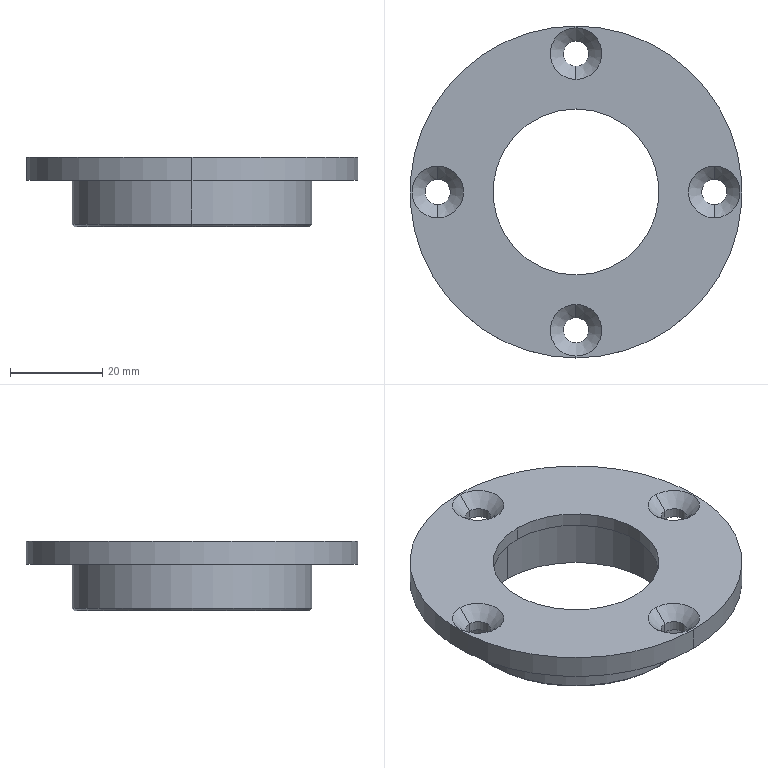Component | SolidWorks | 8TC-A15004-D0-04A-2 | 1 solid | 30 faces | box 72 x 72 x 15 mm | volume 21043 mm3 | cylinder 16 | cone 10 | plane 4 | commonest cylinder face diameters 5.5 x8 42 x2 52 x2 72 x2 36 x2 | material A3
build123d program:
from build123d import *

# Parameters (mm, degrees)
CHAMFER1_SIZE                                        = 0.5
M5_HEX_SOCKET_COUNTERSUNK_HEAD_SCREW_TAP_D           = 5.5
M5_HEX_SOCKET_COUNTERSUNK_HEAD_SCREW_TAP_CSINK_D     = 11.2
M5_HEX_SOCKET_COUNTERSUNK_HEAD_SCREW_TAP_CSINK_ANGLE = 90
CIRPATTERN1_COUNT                                    = 4


with BuildPart() as part:
    # Sketch1 → Revolve1 (revolve)
    with BuildSketch(Plane(origin=(0, 0, 0), x_dir=(1, 0, 0), z_dir=(0, 1, 0)), mode=Mode.PRIVATE) as revolve1_sk:
        Polygon((-18, 0), (-36, 0), (-36, 5), (-26, 5), (-26, 15), (-21, 15), (-21, 3), (-18, 3), align=None)
    revolve(revolve1_sk.sketch.rotate(Axis((0, 0, 0), (0, 0, -1)), 180), axis=Axis((0, 0, 0), (0, 0, -1)))

    # Chamfer1
    chamfer1_edges = [part.edges().sort_by_distance(p)[0] for p in [
        (-26, 0, -15),
    ]]
    chamfer(chamfer1_edges, length=CHAMFER1_SIZE)

    # M5 Hex Socket Countersunk Head Screw Tap (through all)
    with Locations(Plane.XY):
        with Locations((0, 30)):
            m5_hex_socket_countersunk_head_screw_tap = CounterSinkHole(M5_HEX_SOCKET_COUNTERSUNK_HEAD_SCREW_TAP_D / 2, M5_HEX_SOCKET_COUNTERSUNK_HEAD_SCREW_TAP_CSINK_D / 2, counter_sink_angle=M5_HEX_SOCKET_COUNTERSUNK_HEAD_SCREW_TAP_CSINK_ANGLE)

    # CirPattern1: M5 Hex Socket Countersunk Head Screw Tap ×4 about axis
    cirpattern1_axis = Axis((0, 0, 0), (0, 0, 1))
    for i in range(1, CIRPATTERN1_COUNT):
        add(m5_hex_socket_countersunk_head_screw_tap.rotate(cirpattern1_axis, i * 360 / CIRPATTERN1_COUNT), mode=Mode.SUBTRACT)


solid = part.part

# Placed as in the assembly
solid = solid.moved(Location((-7.5, 234.5, 125), (0, 0, 0)))
STEP:
#1=COLOUR_RGB('',0.7922,0.8196,0.9333);
#2=FILL_AREA_STYLE_COLOUR('',#1);
#3=FILL_AREA_STYLE('',(#2));
#4=SURFACE_STYLE_FILL_AREA(#3);
#5=SURFACE_SIDE_STYLE('',(#4));
#6=SURFACE_STYLE_USAGE(.BOTH.,#5);
#7=PRESENTATION_STYLE_ASSIGNMENT((#6));
#8=CARTESIAN_POINT('',(-0.2953,10.305,4.809));
#9=VERTEX_POINT('',#8);
#10=CARTESIAN_POINT('',(-0.2953,10.522,4.809));
#11=VERTEX_POINT('',#10);
#12=CARTESIAN_POINT('',(-0.2953,10.413,4.809));
#13=DIRECTION('',(0.,0.,1.));
#14=DIRECTION('',(0.,1.,0.));
#15=AXIS2_PLACEMENT_3D('',#12,#13,#14);
#16=CIRCLE('',#15,0.1083);
#17=EDGE_CURVE('',#9,#11,#16,.T.);
#18=ORIENTED_EDGE('',*,*,#17,.F.);
#19=CARTESIAN_POINT('',(-0.2953,10.193,4.921));
#20=VERTEX_POINT('',#19);
#21=CARTESIAN_POINT('',(-0.2953,10.193,4.921));
#22=DIRECTION('',(-0.,-0.7071,0.7071));
#23=VECTOR('',#22,39.37);
#24=LINE('',#21,#23);
#25=EDGE_CURVE('',#9,#20,#24,.T.);
#26=ORIENTED_EDGE('',*,*,#25,.T.);
#27=CARTESIAN_POINT('',(-0.2953,10.634,4.921));
#28=VERTEX_POINT('',#27);
#29=CARTESIAN_POINT('',(-0.2953,10.413,4.921));
#30=DIRECTION('',(0.,0.,1.));
#31=DIRECTION('',(0.,1.,0.));
#32=AXIS2_PLACEMENT_3D('',#29,#30,#31);
#33=CIRCLE('',#32,0.2205);
#34=EDGE_CURVE('',#20,#28,#33,.T.);
#35=ORIENTED_EDGE('',*,*,#34,.T.);
#36=CARTESIAN_POINT('',(-0.2953,10.634,4.921));
#37=DIRECTION('',(0.,0.7071,0.7071));
#38=VECTOR('',#37,39.37);
#39=LINE('',#36,#38);
#40=EDGE_CURVE('',#11,#28,#39,.T.);
#41=ORIENTED_EDGE('',*,*,#40,.F.);
#42=EDGE_LOOP('',(#18,#26,#35,#41));
#43=FACE_OUTER_BOUND('',#42,.T.);
#44=CARTESIAN_POINT('',(-0.2953,10.413,4.921));
#45=DIRECTION('',(0.,0.,1.));
#46=DIRECTION('',(0.,1.,0.));
#47=AXIS2_PLACEMENT_3D('',#44,#45,#46);
#48=CONICAL_SURFACE('',#47,0.2205,0.7854);
#49=ADVANCED_FACE('',(#43),#48,.F.);
#50=CARTESIAN_POINT('',(-0.2953,10.305,4.724));
#51=VERTEX_POINT('',#50);
#52=CARTESIAN_POINT('',(-0.2953,10.522,4.724));
#53=VERTEX_POINT('',#52);
#54=CARTESIAN_POINT('',(-0.2953,10.413,4.724));
#55=DIRECTION('',(0.,0.,1.));
#56=DIRECTION('',(0.,1.,0.));
#57=AXIS2_PLACEMENT_3D('',#54,#55,#56);
#58=CIRCLE('',#57,0.1083);
#59=EDGE_CURVE('',#51,#53,#58,.T.);
#60=ORIENTED_EDGE('',*,*,#59,.F.);
#61=CARTESIAN_POINT('',(-0.2953,10.305,4.921));
#62=DIRECTION('',(0.,0.,1.));
#63=VECTOR('',#62,39.37);
#64=LINE('',#61,#63);
#65=EDGE_CURVE('',#51,#9,#64,.T.);
#66=ORIENTED_EDGE('',*,*,#65,.T.);
#67=ORIENTED_EDGE('',*,*,#17,.T.);
#68=CARTESIAN_POINT('',(-0.2953,10.522,4.921));
#69=DIRECTION('',(0.,0.,1.));
#70=VECTOR('',#69,39.37);
#71=LINE('',#68,#70);
#72=EDGE_CURVE('',#53,#11,#71,.T.);
#73=ORIENTED_EDGE('',*,*,#72,.F.);
#74=EDGE_LOOP('',(#60,#66,#67,#73));
#75=FACE_OUTER_BOUND('',#74,.T.);
#76=CARTESIAN_POINT('',(-0.2953,10.413,4.921));
#77=DIRECTION('',(0.,0.,1.));
#78=DIRECTION('',(0.,1.,0.));
#79=AXIS2_PLACEMENT_3D('',#76,#77,#78);
#80=CYLINDRICAL_SURFACE('',#79,0.1083);
#81=ADVANCED_FACE('',(#75),#80,.F.);
#82=CARTESIAN_POINT('',(0.8858,9.124,4.809));
#83=VERTEX_POINT('',#82);
#84=CARTESIAN_POINT('',(0.8858,9.341,4.809));
#85=VERTEX_POINT('',#84);
#86=CARTESIAN_POINT('',(0.8858,9.232,4.809));
#87=DIRECTION('',(0.,0.,1.));
#88=DIRECTION('',(0.,1.,0.));
#89=AXIS2_PLACEMENT_3D('',#86,#87,#88);
#90=CIRCLE('',#89,0.1083);
#91=EDGE_CURVE('',#83,#85,#90,.T.);
#92=ORIENTED_EDGE('',*,*,#91,.F.);
#93=CARTESIAN_POINT('',(0.8858,9.012,4.921));
#94=VERTEX_POINT('',#93);
#95=CARTESIAN_POINT('',(0.8858,9.012,4.921));
#96=DIRECTION('',(-0.,-0.7071,0.7071));
#97=VECTOR('',#96,39.37);
#98=LINE('',#95,#97);
#99=EDGE_CURVE('',#83,#94,#98,.T.);
#100=ORIENTED_EDGE('',*,*,#99,.T.);
#101=CARTESIAN_POINT('',(0.8858,9.453,4.921));
#102=VERTEX_POINT('',#101);
#103=CARTESIAN_POINT('',(0.8858,9.232,4.921));
#104=DIRECTION('',(0.,0.,1.));
#105=DIRECTION('',(0.,1.,0.));
#106=AXIS2_PLACEMENT_3D('',#103,#104,#105);
#107=CIRCLE('',#106,0.2205);
#108=EDGE_CURVE('',#94,#102,#107,.T.);
#109=ORIENTED_EDGE('',*,*,#108,.T.);
#110=CARTESIAN_POINT('',(0.8858,9.453,4.921));
#111=DIRECTION('',(0.,0.7071,0.7071));
#112=VECTOR('',#111,39.37);
#113=LINE('',#110,#112);
#114=EDGE_CURVE('',#85,#102,#113,.T.);
#115=ORIENTED_EDGE('',*,*,#114,.F.);
#116=EDGE_LOOP('',(#92,#100,#109,#115));
#117=FACE_OUTER_BOUND('',#116,.T.);
#118=CARTESIAN_POINT('',(0.8858,9.232,4.921));
#119=DIRECTION('',(0.,0.,1.));
#120=DIRECTION('',(0.,1.,0.));
#121=AXIS2_PLACEMENT_3D('',#118,#119,#120);
#122=CONICAL_SURFACE('',#121,0.2205,0.7854);
#123=ADVANCED_FACE('',(#117),#122,.F.);
#124=CARTESIAN_POINT('',(0.8858,9.124,4.724));
#125=VERTEX_POINT('',#124);
#126=CARTESIAN_POINT('',(0.8858,9.341,4.724));
#127=VERTEX_POINT('',#126);
#128=CARTESIAN_POINT('',(0.8858,9.232,4.724));
#129=DIRECTION('',(0.,0.,1.));
#130=DIRECTION('',(0.,1.,0.));
#131=AXIS2_PLACEMENT_3D('',#128,#129,#130);
#132=CIRCLE('',#131,0.1083);
#133=EDGE_CURVE('',#125,#127,#132,.T.);
#134=ORIENTED_EDGE('',*,*,#133,.F.);
#135=CARTESIAN_POINT('',(0.8858,9.124,4.921));
#136=DIRECTION('',(0.,0.,1.));
#137=VECTOR('',#136,39.37);
#138=LINE('',#135,#137);
#139=EDGE_CURVE('',#125,#83,#138,.T.);
#140=ORIENTED_EDGE('',*,*,#139,.T.);
#141=ORIENTED_EDGE('',*,*,#91,.T.);
#142=CARTESIAN_POINT('',(0.8858,9.341,4.921));
#143=DIRECTION('',(0.,0.,1.));
#144=VECTOR('',#143,39.37);
#145=LINE('',#142,#144);
#146=EDGE_CURVE('',#127,#85,#145,.T.);
#147=ORIENTED_EDGE('',*,*,#146,.F.);
#148=EDGE_LOOP('',(#134,#140,#141,#147));
#149=FACE_OUTER_BOUND('',#148,.T.);
#150=CARTESIAN_POINT('',(0.8858,9.232,4.921));
#151=DIRECTION('',(0.,0.,1.));
#152=DIRECTION('',(0.,1.,0.));
#153=AXIS2_PLACEMENT_3D('',#150,#151,#152);
#154=CYLINDRICAL_SURFACE('',#153,0.1083);
#155=ADVANCED_FACE('',(#149),#154,.F.);
#156=CARTESIAN_POINT('',(-0.2953,7.943,4.809));
#157=VERTEX_POINT('',#156);
#158=CARTESIAN_POINT('',(-0.2953,8.159,4.809));
#159=VERTEX_POINT('',#158);
#160=CARTESIAN_POINT('',(-0.2953,8.051,4.809));
#161=DIRECTION('',(0.,0.,1.));
#162=DIRECTION('',(0.,1.,0.));
#163=AXIS2_PLACEMENT_3D('',#160,#161,#162);
#164=CIRCLE('',#163,0.1083);
#165=EDGE_CURVE('',#157,#159,#164,.T.);
#166=ORIENTED_EDGE('',*,*,#165,.F.);
#167=CARTESIAN_POINT('',(-0.2953,7.831,4.921));
#168=VERTEX_POINT('',#167);
#169=CARTESIAN_POINT('',(-0.2953,7.831,4.921));
#170=DIRECTION('',(-0.,-0.7071,0.7071));
#171=VECTOR('',#170,39.37);
#172=LINE('',#169,#171);
#173=EDGE_CURVE('',#157,#168,#172,.T.);
#174=ORIENTED_EDGE('',*,*,#173,.T.);
#175=CARTESIAN_POINT('',(-0.2953,8.272,4.921));
#176=VERTEX_POINT('',#175);
#177=CARTESIAN_POINT('',(-0.2953,8.051,4.921));
#178=DIRECTION('',(0.,0.,1.));
#179=DIRECTION('',(0.,1.,0.));
#180=AXIS2_PLACEMENT_3D('',#177,#178,#179);
#181=CIRCLE('',#180,0.2205);
#182=EDGE_CURVE('',#168,#176,#181,.T.);
#183=ORIENTED_EDGE('',*,*,#182,.T.);
#184=CARTESIAN_POINT('',(-0.2953,8.272,4.921));
#185=DIRECTION('',(0.,0.7071,0.7071));
#186=VECTOR('',#185,39.37);
#187=LINE('',#184,#186);
#188=EDGE_CURVE('',#159,#176,#187,.T.);
#189=ORIENTED_EDGE('',*,*,#188,.F.);
#190=EDGE_LOOP('',(#166,#174,#183,#189));
#191=FACE_OUTER_BOUND('',#190,.T.);
#192=CARTESIAN_POINT('',(-0.2953,8.051,4.921));
#193=DIRECTION('',(0.,0.,1.));
#194=DIRECTION('',(0.,1.,0.));
#195=AXIS2_PLACEMENT_3D('',#192,#193,#194);
#196=CONICAL_SURFACE('',#195,0.2205,0.7854);
#197=ADVANCED_FACE('',(#191),#196,.F.);
#198=CARTESIAN_POINT('',(-0.2953,7.943,4.724));
#199=VERTEX_POINT('',#198);
#200=CARTESIAN_POINT('',(-0.2953,8.159,4.724));
#201=VERTEX_POINT('',#200);
#202=CARTESIAN_POINT('',(-0.2953,8.051,4.724));
#203=DIRECTION('',(0.,0.,1.));
#204=DIRECTION('',(0.,1.,0.));
#205=AXIS2_PLACEMENT_3D('',#202,#203,#204);
#206=CIRCLE('',#205,0.1083);
#207=EDGE_CURVE('',#199,#201,#206,.T.);
#208=ORIENTED_EDGE('',*,*,#207,.F.);
#209=CARTESIAN_POINT('',(-0.2953,7.943,4.921));
#210=DIRECTION('',(0.,0.,1.));
#211=VECTOR('',#210,39.37);
#212=LINE('',#209,#211);
#213=EDGE_CURVE('',#199,#157,#212,.T.);
#214=ORIENTED_EDGE('',*,*,#213,.T.);
#215=ORIENTED_EDGE('',*,*,#165,.T.);
#216=CARTESIAN_POINT('',(-0.2953,8.159,4.921));
#217=DIRECTION('',(0.,0.,1.));
#218=VECTOR('',#217,39.37);
#219=LINE('',#216,#218);
#220=EDGE_CURVE('',#201,#159,#219,.T.);
#221=ORIENTED_EDGE('',*,*,#220,.F.);
#222=EDGE_LOOP('',(#208,#214,#215,#221));
#223=FACE_OUTER_BOUND('',#222,.T.);
#224=CARTESIAN_POINT('',(-0.2953,8.051,4.921));
#225=DIRECTION('',(0.,0.,1.));
#226=DIRECTION('',(0.,1.,0.));
#227=AXIS2_PLACEMENT_3D('',#224,#225,#226);
#228=CYLINDRICAL_SURFACE('',#227,0.1083);
#229=ADVANCED_FACE('',(#223),#228,.F.);
#230=CARTESIAN_POINT('',(-1.476,9.124,4.809));
#231=VERTEX_POINT('',#230);
#232=CARTESIAN_POINT('',(-1.476,9.341,4.809));
#233=VERTEX_POINT('',#232);
#234=CARTESIAN_POINT('',(-1.476,9.232,4.809));
#235=DIRECTION('',(0.,0.,1.));
#236=DIRECTION('',(0.,1.,0.));
#237=AXIS2_PLACEMENT_3D('',#234,#235,#236);
#238=CIRCLE('',#237,0.1083);
#239=EDGE_CURVE('',#231,#233,#238,.T.);
#240=ORIENTED_EDGE('',*,*,#239,.F.);
#241=CARTESIAN_POINT('',(-1.476,9.012,4.921));
#242=VERTEX_POINT('',#241);
#243=CARTESIAN_POINT('',(-1.476,9.012,4.921));
#244=DIRECTION('',(-0.,-0.7071,0.7071));
#245=VECTOR('',#244,39.37);
#246=LINE('',#243,#245);
#247=EDGE_CURVE('',#231,#242,#246,.T.);
#248=ORIENTED_EDGE('',*,*,#247,.T.);
#249=CARTESIAN_POINT('',(-1.476,9.453,4.921));
#250=VERTEX_POINT('',#249);
#251=CARTESIAN_POINT('',(-1.476,9.232,4.921));
#252=DIRECTION('',(0.,0.,1.));
#253=DIRECTION('',(0.,1.,0.));
#254=AXIS2_PLACEMENT_3D('',#251,#252,#253);
#255=CIRCLE('',#254,0.2205);
#256=EDGE_CURVE('',#242,#250,#255,.T.);
#257=ORIENTED_EDGE('',*,*,#256,.T.);
#258=CARTESIAN_POINT('',(-1.476,9.453,4.921));
#259=DIRECTION('',(0.,0.7071,0.7071));
#260=VECTOR('',#259,39.37);
#261=LINE('',#258,#260);
#262=EDGE_CURVE('',#233,#250,#261,.T.);
#263=ORIENTED_EDGE('',*,*,#262,.F.);
#264=EDGE_LOOP('',(#240,#248,#257,#263));
#265=FACE_OUTER_BOUND('',#264,.T.);
#266=CARTESIAN_POINT('',(-1.476,9.232,4.921));
#267=DIRECTION('',(0.,0.,1.));
#268=DIRECTION('',(0.,1.,0.));
#269=AXIS2_PLACEMENT_3D('',#266,#267,#268);
#270=CONICAL_SURFACE('',#269,0.2205,0.7854);
#271=ADVANCED_FACE('',(#265),#270,.F.);
#272=CARTESIAN_POINT('',(-1.476,9.124,4.724));
#273=VERTEX_POINT('',#272);
#274=CARTESIAN_POINT('',(-1.476,9.341,4.724));
#275=VERTEX_POINT('',#274);
#276=CARTESIAN_POINT('',(-1.476,9.232,4.724));
#277=DIRECTION('',(0.,0.,1.));
#278=DIRECTION('',(0.,1.,0.));
#279=AXIS2_PLACEMENT_3D('',#276,#277,#278);
#280=CIRCLE('',#279,0.1083);
#281=EDGE_CURVE('',#273,#275,#280,.T.);
#282=ORIENTED_EDGE('',*,*,#281,.F.);
#283=CARTESIAN_POINT('',(-1.476,9.124,4.921));
#284=DIRECTION('',(0.,0.,1.));
#285=VECTOR('',#284,39.37);
#286=LINE('',#283,#285);
#287=EDGE_CURVE('',#273,#231,#286,.T.);
#288=ORIENTED_EDGE('',*,*,#287,.T.);
#289=ORIENTED_EDGE('',*,*,#239,.T.);
#290=CARTESIAN_POINT('',(-1.476,9.341,4.921));
#291=DIRECTION('',(0.,0.,1.));
#292=VECTOR('',#291,39.37);
#293=LINE('',#290,#292);
#294=EDGE_CURVE('',#275,#233,#293,.T.);
#295=ORIENTED_EDGE('',*,*,#294,.F.);
#296=EDGE_LOOP('',(#282,#288,#289,#295));
#297=FACE_OUTER_BOUND('',#296,.T.);
#298=CARTESIAN_POINT('',(-1.476,9.232,4.921));
#299=DIRECTION('',(0.,0.,1.));
#300=DIRECTION('',(0.,1.,0.));
#301=AXIS2_PLACEMENT_3D('',#298,#299,#300);
#302=CYLINDRICAL_SURFACE('',#301,0.1083);
#303=ADVANCED_FACE('',(#297),#302,.F.);
#304=CARTESIAN_POINT('',(-0.2953,8.228,4.331));
#305=VERTEX_POINT('',#304);
#306=CARTESIAN_POINT('',(-0.2953,10.236,4.331));
#307=VERTEX_POINT('',#306);
#308=CARTESIAN_POINT('',(-0.2953,9.232,4.331));
#309=DIRECTION('',(0.,0.,-1.));
#310=DIRECTION('',(0.,1.,0.));
#311=AXIS2_PLACEMENT_3D('',#308,#309,#310);
#312=CIRCLE('',#311,1.004);
#313=EDGE_CURVE('',#305,#307,#312,.T.);
#314=ORIENTED_EDGE('',*,*,#313,.F.);
#315=CARTESIAN_POINT('',(-0.2953,8.209,4.35));
#316=VERTEX_POINT('',#315);
#317=CARTESIAN_POINT('',(-0.2953,8.209,4.35));
#318=DIRECTION('',(-0.,-0.7071,0.7071));
#319=VECTOR('',#318,39.37);
#320=LINE('',#317,#319);
#321=EDGE_CURVE('',#305,#316,#320,.T.);
#322=ORIENTED_EDGE('',*,*,#321,.T.);
#323=CARTESIAN_POINT('',(-0.2953,10.256,4.35));
#324=VERTEX_POINT('',#323);
#325=CARTESIAN_POINT('',(-0.2953,9.232,4.35));
#326=DIRECTION('',(0.,0.,1.));
#327=DIRECTION('',(0.,1.,0.));
#328=AXIS2_PLACEMENT_3D('',#325,#326,#327);
#329=CIRCLE('',#328,1.024);
#330=EDGE_CURVE('',#324,#316,#329,.T.);
#331=ORIENTED_EDGE('',*,*,#330,.F.);
#332=CARTESIAN_POINT('',(-0.2953,10.256,4.35));
#333=DIRECTION('',(0.,0.7071,0.7071));
#334=VECTOR('',#333,39.37);
#335=LINE('',#332,#334);
#336=EDGE_CURVE('',#307,#324,#335,.T.);
#337=ORIENTED_EDGE('',*,*,#336,.F.);
#338=EDGE_LOOP('',(#314,#322,#331,#337));
#339=FACE_OUTER_BOUND('',#338,.T.);
#340=CARTESIAN_POINT('',(-0.2953,9.232,4.35));
#341=DIRECTION('',(0.,0.,1.));
#342=DIRECTION('',(0.,1.,0.));
#343=AXIS2_PLACEMENT_3D('',#340,#341,#342);
#344=CONICAL_SURFACE('',#343,1.024,0.7854);
#345=ADVANCED_FACE('',(#339),#344,.T.);
#346=CARTESIAN_POINT('',(-0.2953,8.406,4.331));
#347=VERTEX_POINT('',#346);
#348=CARTESIAN_POINT('',(-0.2953,10.059,4.331));
#349=VERTEX_POINT('',#348);
#350=CARTESIAN_POINT('',(-0.2953,9.232,4.331));
#351=DIRECTION('',(0.,0.,1.));
#352=DIRECTION('',(0.,1.,0.));
#353=AXIS2_PLACEMENT_3D('',#350,#351,#352);
#354=CIRCLE('',#353,0.8268);
#355=EDGE_CURVE('',#347,#349,#354,.T.);
#356=ORIENTED_EDGE('',*,*,#355,.F.);
#357=CARTESIAN_POINT('',(-0.2953,8.406,4.803));
#358=VERTEX_POINT('',#357);
#359=CARTESIAN_POINT('',(-0.2953,8.406,4.921));
#360=DIRECTION('',(0.,0.,1.));
#361=VECTOR('',#360,39.37);
#362=LINE('',#359,#361);
#363=EDGE_CURVE('',#347,#358,#362,.T.);
#364=ORIENTED_EDGE('',*,*,#363,.T.);
#365=CARTESIAN_POINT('',(-0.2953,10.059,4.803));
#366=VERTEX_POINT('',#365);
#367=CARTESIAN_POINT('',(-0.2953,9.232,4.803));
#368=DIRECTION('',(0.,0.,1.));
#369=DIRECTION('',(0.,1.,0.));
#370=AXIS2_PLACEMENT_3D('',#367,#368,#369);
#371=CIRCLE('',#370,0.8268);
#372=EDGE_CURVE('',#358,#366,#371,.T.);
#373=ORIENTED_EDGE('',*,*,#372,.T.);
#374=CARTESIAN_POINT('',(-0.2953,10.059,4.921));
#375=DIRECTION('',(0.,0.,1.));
#376=VECTOR('',#375,39.37);
#377=LINE('',#374,#376);
#378=EDGE_CURVE('',#349,#366,#377,.T.);
#379=ORIENTED_EDGE('',*,*,#378,.F.);
#380=EDGE_LOOP('',(#356,#364,#373,#379));
#381=FACE_OUTER_BOUND('',#380,.T.);
#382=CARTESIAN_POINT('',(-0.2953,9.232,4.921));
#383=DIRECTION('',(0.,0.,1.));
#384=DIRECTION('',(0.,1.,0.));
#385=AXIS2_PLACEMENT_3D('',#382,#383,#384);
#386=CYLINDRICAL_SURFACE('',#385,0.8268);
#387=ADVANCED_FACE('',(#381),#386,.F.);
#388=ORIENTED_EDGE('',*,*,#330,.T.);
#389=CARTESIAN_POINT('',(-0.2953,8.209,4.724));
#390=VERTEX_POINT('',#389);
#391=CARTESIAN_POINT('',(-0.2953,8.209,4.921));
#392=DIRECTION('',(0.,0.,1.));
#393=VECTOR('',#392,39.37);
#394=LINE('',#391,#393);
#395=EDGE_CURVE('',#316,#390,#394,.T.);
#396=ORIENTED_EDGE('',*,*,#395,.T.);
#397=CARTESIAN_POINT('',(-0.2953,10.256,4.724));
#398=VERTEX_POINT('',#397);
#399=CARTESIAN_POINT('',(-0.2953,9.232,4.724));
#400=DIRECTION('',(0.,0.,1.));
#401=DIRECTION('',(0.,1.,0.));
#402=AXIS2_PLACEMENT_3D('',#399,#400,#401);
#403=CIRCLE('',#402,1.024);
#404=EDGE_CURVE('',#398,#390,#403,.T.);
#405=ORIENTED_EDGE('',*,*,#404,.F.);
#406=CARTESIAN_POINT('',(-0.2953,10.256,4.921));
#407=DIRECTION('',(0.,0.,1.));
#408=VECTOR('',#407,39.37);
#409=LINE('',#406,#408);
#410=EDGE_CURVE('',#324,#398,#409,.T.);
#411=ORIENTED_EDGE('',*,*,#410,.F.);
#412=EDGE_LOOP('',(#388,#396,#405,#411));
#413=FACE_OUTER_BOUND('',#412,.T.);
#414=CARTESIAN_POINT('',(-0.2953,9.232,4.921));
#415=DIRECTION('',(0.,0.,1.));
#416=DIRECTION('',(0.,1.,0.));
#417=AXIS2_PLACEMENT_3D('',#414,#415,#416);
#418=CYLINDRICAL_SURFACE('',#417,1.024);
#419=ADVANCED_FACE('',(#413),#418,.T.);
#420=CARTESIAN_POINT('',(-0.2953,10.65,4.724));
#421=VERTEX_POINT('',#420);
#422=CARTESIAN_POINT('',(-0.2953,7.815,4.724));
#423=VERTEX_POINT('',#422);
#424=CARTESIAN_POINT('',(-0.2953,9.232,4.724));
#425=DIRECTION('',(0.,0.,1.));
#426=DIRECTION('',(0.,1.,0.));
#427=AXIS2_PLACEMENT_3D('',#424,#425,#426);
#428=CIRCLE('',#427,1.417);
#429=EDGE_CURVE('',#421,#423,#428,.T.);
#430=ORIENTED_EDGE('',*,*,#429,.T.);
#431=CARTESIAN_POINT('',(-0.2953,7.815,4.921));
#432=VERTEX_POINT('',#431);
#433=CARTESIAN_POINT('',(-0.2953,7.815,4.921));
#434=DIRECTION('',(0.,0.,1.));
#435=VECTOR('',#434,39.37);
#436=LINE('',#433,#435);
#437=EDGE_CURVE('',#423,#432,#436,.T.);
#438=ORIENTED_EDGE('',*,*,#437,.T.);
#439=CARTESIAN_POINT('',(-0.2953,10.65,4.921));
#440=VERTEX_POINT('',#439);
#441=CARTESIAN_POINT('',(-0.2953,9.232,4.921));
#442=DIRECTION('',(0.,0.,1.));
#443=DIRECTION('',(0.,1.,0.));
#444=AXIS2_PLACEMENT_3D('',#441,#442,#443);
#445=CIRCLE('',#444,1.417);
#446=EDGE_CURVE('',#440,#432,#445,.T.);
#447=ORIENTED_EDGE('',*,*,#446,.F.);
#448=CARTESIAN_POINT('',(-0.2953,10.65,4.921));
#449=DIRECTION('',(0.,0.,1.));
#450=VECTOR('',#449,39.37);
#451=LINE('',#448,#450);
#452=EDGE_CURVE('',#421,#440,#451,.T.);
#453=ORIENTED_EDGE('',*,*,#452,.F.);
#454=EDGE_LOOP('',(#430,#438,#447,#453));
#455=FACE_OUTER_BOUND('',#454,.T.);
#456=CARTESIAN_POINT('',(-0.2953,9.232,4.921));
#457=DIRECTION('',(0.,0.,1.));
#458=DIRECTION('',(0.,1.,0.));
#459=AXIS2_PLACEMENT_3D('',#456,#457,#458);
#460=CYLINDRICAL_SURFACE('',#459,1.417);
#461=ADVANCED_FACE('',(#455),#460,.T.);
#462=CARTESIAN_POINT('',(-0.2953,8.524,4.803));
#463=VERTEX_POINT('',#462);
#464=CARTESIAN_POINT('',(-0.2953,9.941,4.803));
#465=VERTEX_POINT('',#464);
#466=CARTESIAN_POINT('',(-0.2953,9.232,4.803));
#467=DIRECTION('',(0.,0.,1.));
#468=DIRECTION('',(0.,1.,0.));
#469=AXIS2_PLACEMENT_3D('',#466,#467,#468);
#470=CIRCLE('',#469,0.7087);
#471=EDGE_CURVE('',#463,#465,#470,.T.);
#472=ORIENTED_EDGE('',*,*,#471,.F.);
#473=CARTESIAN_POINT('',(-0.2953,8.524,4.921));
#474=VERTEX_POINT('',#473);
#475=CARTESIAN_POINT('',(-0.2953,8.524,4.921));
#476=DIRECTION('',(0.,0.,1.));
#477=VECTOR('',#476,39.37);
#478=LINE('',#475,#477);
#479=EDGE_CURVE('',#463,#474,#478,.T.);
#480=ORIENTED_EDGE('',*,*,#479,.T.);
#481=CARTESIAN_POINT('',(-0.2953,9.941,4.921));
#482=VERTEX_POINT('',#481);
#483=CARTESIAN_POINT('',(-0.2953,9.232,4.921));
#484=DIRECTION('',(0.,0.,1.));
#485=DIRECTION('',(0.,1.,0.));
#486=AXIS2_PLACEMENT_3D('',#483,#484,#485);
#487=CIRCLE('',#486,0.7087);
#488=EDGE_CURVE('',#474,#482,#487,.T.);
#489=ORIENTED_EDGE('',*,*,#488,.T.);
#490=CARTESIAN_POINT('',(-0.2953,9.941,4.921));
#491=DIRECTION('',(0.,0.,1.));
#492=VECTOR('',#491,39.37);
#493=LINE('',#490,#492);
#494=EDGE_CURVE('',#465,#482,#493,.T.);
#495=ORIENTED_EDGE('',*,*,#494,.F.);
#496=EDGE_LOOP('',(#472,#480,#489,#495));
#497=FACE_OUTER_BOUND('',#496,.T.);
#498=CARTESIAN_POINT('',(-0.2953,9.232,4.921));
#499=DIRECTION('',(0.,0.,1.));
#500=DIRECTION('',(0.,1.,0.));
#501=AXIS2_PLACEMENT_3D('',#498,#499,#500);
#502=CYLINDRICAL_SURFACE('',#501,0.7087);
#503=ADVANCED_FACE('',(#497),#502,.F.);
#504=ORIENTED_EDGE('',*,*,#479,.F.);
#505=CARTESIAN_POINT('',(-0.2953,9.232,4.803));
#506=DIRECTION('',(0.,0.,1.));
#507=DIRECTION('',(0.,1.,0.));
#508=AXIS2_PLACEMENT_3D('',#505,#506,#507);
#509=CIRCLE('',#508,0.7087);
#510=EDGE_CURVE('',#465,#463,#509,.T.);
#511=ORIENTED_EDGE('',*,*,#510,.F.);
#512=ORIENTED_EDGE('',*,*,#494,.T.);
#513=CARTESIAN_POINT('',(-0.2953,9.232,4.921));
#514=DIRECTION('',(0.,0.,1.));
#515=DIRECTION('',(0.,1.,0.));
#516=AXIS2_PLACEMENT_3D('',#513,#514,#515);
#517=CIRCLE('',#516,0.7087);
#518=EDGE_CURVE('',#482,#474,#517,.T.);
#519=ORIENTED_EDGE('',*,*,#518,.T.);
#520=EDGE_LOOP('',(#504,#511,#512,#519));
#521=FACE_OUTER_BOUND('',#520,.T.);
#522=CARTESIAN_POINT('',(-0.2953,9.232,4.921));
#523=DIRECTION('',(0.,0.,1.));
#524=DIRECTION('',(0.,1.,0.));
#525=AXIS2_PLACEMENT_3D('',#522,#523,#524);
#526=CYLINDRICAL_SURFACE('',#525,0.7087);
#527=ADVANCED_FACE('',(#521),#526,.F.);
#528=CARTESIAN_POINT('',(-0.2953,10.413,4.921));
#529=DIRECTION('',(0.,0.,1.));
#530=DIRECTION('',(0.,1.,0.));
#531=AXIS2_PLACEMENT_3D('',#528,#529,#530);
#532=CIRCLE('',#531,0.2205);
#533=EDGE_CURVE('',#28,#20,#532,.T.);
#534=ORIENTED_EDGE('',*,*,#533,.F.);
#535=ORIENTED_EDGE('',*,*,#34,.F.);
#536=EDGE_LOOP('',(#534,#535));
#537=FACE_BOUND('',#536,.T.);
#538=CARTESIAN_POINT('',(0.8858,9.232,4.921));
#539=DIRECTION('',(0.,0.,1.));
#540=DIRECTION('',(0.,1.,0.));
#541=AXIS2_PLACEMENT_3D('',#538,#539,#540);
#542=CIRCLE('',#541,0.2205);
#543=EDGE_CURVE('',#102,#94,#542,.T.);
#544=ORIENTED_EDGE('',*,*,#543,.F.);
#545=ORIENTED_EDGE('',*,*,#108,.F.);
#546=EDGE_LOOP('',(#544,#545));
#547=FACE_BOUND('',#546,.T.);
#548=CARTESIAN_POINT('',(-0.2953,8.051,4.921));
#549=DIRECTION('',(0.,0.,1.));
#550=DIRECTION('',(0.,1.,0.));
#551=AXIS2_PLACEMENT_3D('',#548,#549,#550);
#552=CIRCLE('',#551,0.2205);
#553=EDGE_CURVE('',#176,#168,#552,.T.);
#554=ORIENTED_EDGE('',*,*,#553,.F.);
#555=ORIENTED_EDGE('',*,*,#182,.F.);
#556=EDGE_LOOP('',(#554,#555));
#557=FACE_BOUND('',#556,.T.);
#558=CARTESIAN_POINT('',(-1.476,9.232,4.921));
#559=DIRECTION('',(0.,0.,1.));
#560=DIRECTION('',(0.,1.,0.));
#561=AXIS2_PLACEMENT_3D('',#558,#559,#560);
#562=CIRCLE('',#561,0.2205);
#563=EDGE_CURVE('',#250,#242,#562,.T.);
#564=ORIENTED_EDGE('',*,*,#563,.F.);
#565=ORIENTED_EDGE('',*,*,#256,.F.);
#566=EDGE_LOOP('',(#564,#565));
#567=FACE_BOUND('',#566,.T.);
#568=ORIENTED_EDGE('',*,*,#518,.F.);
#569=ORIENTED_EDGE('',*,*,#488,.F.);
#570=EDGE_LOOP('',(#568,#569));
#571=FACE_BOUND('',#570,.T.);
#572=ORIENTED_EDGE('',*,*,#446,.T.);
#573=CARTESIAN_POINT('',(-0.2953,9.232,4.921));
#574=DIRECTION('',(0.,0.,1.));
#575=DIRECTION('',(0.,1.,0.));
#576=AXIS2_PLACEMENT_3D('',#573,#574,#575);
#577=CIRCLE('',#576,1.417);
#578=EDGE_CURVE('',#432,#440,#577,.T.);
#579=ORIENTED_EDGE('',*,*,#578,.T.);
#580=EDGE_LOOP('',(#572,#579));
#581=FACE_OUTER_BOUND('',#580,.T.);
#582=CARTESIAN_POINT('',(-0.2953,8.524,4.921));
#583=DIRECTION('',(0.,0.,-1.));
#584=DIRECTION('',(-0.,-1.,0.));
#585=AXIS2_PLACEMENT_3D('',#582,#583,#584);
#586=PLANE('',#585);
#587=ADVANCED_FACE('',(#537,#547,#557,#567,#571,#581),#586,.F.);
#588=ORIENTED_EDGE('',*,*,#437,.F.);
#589=CARTESIAN_POINT('',(-0.2953,9.232,4.724));
#590=DIRECTION('',(0.,0.,1.));
#591=DIRECTION('',(0.,1.,0.));
#592=AXIS2_PLACEMENT_3D('',#589,#590,#591);
#593=CIRCLE('',#592,1.417);
#594=EDGE_CURVE('',#423,#421,#593,.T.);
#595=ORIENTED_EDGE('',*,*,#594,.T.);
#596=ORIENTED_EDGE('',*,*,#452,.T.);
#597=ORIENTED_EDGE('',*,*,#578,.F.);
#598=EDGE_LOOP('',(#588,#595,#596,#597));
#599=FACE_OUTER_BOUND('',#598,.T.);
#600=CARTESIAN_POINT('',(-0.2953,9.232,4.921));
#601=DIRECTION('',(0.,0.,1.));
#602=DIRECTION('',(0.,1.,0.));
#603=AXIS2_PLACEMENT_3D('',#600,#601,#602);
#604=CYLINDRICAL_SURFACE('',#603,1.417);
#605=ADVANCED_FACE('',(#599),#604,.T.);
#606=CARTESIAN_POINT('',(-0.2953,10.413,4.724));
#607=DIRECTION('',(0.,0.,1.));
#608=DIRECTION('',(0.,1.,0.));
#609=AXIS2_PLACEMENT_3D('',#606,#607,#608);
#610=CIRCLE('',#609,0.1083);
#611=EDGE_CURVE('',#53,#51,#610,.T.);
#612=ORIENTED_EDGE('',*,*,#611,.T.);
#613=ORIENTED_EDGE('',*,*,#59,.T.);
#614=EDGE_LOOP('',(#612,#613));
#615=FACE_BOUND('',#614,.T.);
#616=CARTESIAN_POINT('',(0.8858,9.232,4.724));
#617=DIRECTION('',(0.,0.,1.));
#618=DIRECTION('',(0.,1.,0.));
#619=AXIS2_PLACEMENT_3D('',#616,#617,#618);
#620=CIRCLE('',#619,0.1083);
#621=EDGE_CURVE('',#127,#125,#620,.T.);
#622=ORIENTED_EDGE('',*,*,#621,.T.);
#623=ORIENTED_EDGE('',*,*,#133,.T.);
#624=EDGE_LOOP('',(#622,#623));
#625=FACE_BOUND('',#624,.T.);
#626=CARTESIAN_POINT('',(-0.2953,8.051,4.724));
#627=DIRECTION('',(0.,0.,1.));
#628=DIRECTION('',(0.,1.,0.));
#629=AXIS2_PLACEMENT_3D('',#626,#627,#628);
#630=CIRCLE('',#629,0.1083);
#631=EDGE_CURVE('',#201,#199,#630,.T.);
#632=ORIENTED_EDGE('',*,*,#631,.T.);
#633=ORIENTED_EDGE('',*,*,#207,.T.);
#634=EDGE_LOOP('',(#632,#633));
#635=FACE_BOUND('',#634,.T.);
#636=CARTESIAN_POINT('',(-1.476,9.232,4.724));
#637=DIRECTION('',(0.,0.,1.));
#638=DIRECTION('',(0.,1.,0.));
#639=AXIS2_PLACEMENT_3D('',#636,#637,#638);
#640=CIRCLE('',#639,0.1083);
#641=EDGE_CURVE('',#275,#273,#640,.T.);
#642=ORIENTED_EDGE('',*,*,#641,.T.);
#643=ORIENTED_EDGE('',*,*,#281,.T.);
#644=EDGE_LOOP('',(#642,#643));
#645=FACE_BOUND('',#644,.T.);
#646=ORIENTED_EDGE('',*,*,#429,.F.);
#647=ORIENTED_EDGE('',*,*,#594,.F.);
#648=EDGE_LOOP('',(#646,#647));
#649=FACE_OUTER_BOUND('',#648,.T.);
#650=ORIENTED_EDGE('',*,*,#404,.T.);
#651=CARTESIAN_POINT('',(-0.2953,9.232,4.724));
#652=DIRECTION('',(0.,0.,1.));
#653=DIRECTION('',(0.,1.,0.));
#654=AXIS2_PLACEMENT_3D('',#651,#652,#653);
#655=CIRCLE('',#654,1.024);
#656=EDGE_CURVE('',#390,#398,#655,.T.);
#657=ORIENTED_EDGE('',*,*,#656,.T.);
#658=EDGE_LOOP('',(#650,#657));
#659=FACE_BOUND('',#658,.T.);
#660=CARTESIAN_POINT('',(-0.2953,7.815,4.724));
#661=DIRECTION('',(0.,0.,1.));
#662=DIRECTION('',(0.,1.,0.));
#663=AXIS2_PLACEMENT_3D('',#660,#661,#662);
#664=PLANE('',#663);
#665=ADVANCED_FACE('',(#615,#625,#635,#645,#649,#659),#664,.F.);
#666=ORIENTED_EDGE('',*,*,#395,.F.);
#667=CARTESIAN_POINT('',(-0.2953,9.232,4.35));
#668=DIRECTION('',(0.,0.,1.));
#669=DIRECTION('',(0.,1.,0.));
#670=AXIS2_PLACEMENT_3D('',#667,#668,#669);
#671=CIRCLE('',#670,1.024);
#672=EDGE_CURVE('',#316,#324,#671,.T.);
#673=ORIENTED_EDGE('',*,*,#672,.T.);
#674=ORIENTED_EDGE('',*,*,#410,.T.);
#675=ORIENTED_EDGE('',*,*,#656,.F.);
#676=EDGE_LOOP('',(#666,#673,#674,#675));
#677=FACE_OUTER_BOUND('',#676,.T.);
#678=CARTESIAN_POINT('',(-0.2953,9.232,4.921));
#679=DIRECTION('',(0.,0.,1.));
#680=DIRECTION('',(0.,1.,0.));
#681=AXIS2_PLACEMENT_3D('',#678,#679,#680);
#682=CYLINDRICAL_SURFACE('',#681,1.024);
#683=ADVANCED_FACE('',(#677),#682,.T.);
#684=CARTESIAN_POINT('',(-0.2953,9.232,4.331));
#685=DIRECTION('',(0.,0.,-1.));
#686=DIRECTION('',(0.,1.,0.));
#687=AXIS2_PLACEMENT_3D('',#684,#685,#686);
#688=CIRCLE('',#687,1.004);
#689=EDGE_CURVE('',#307,#305,#688,.T.);
#690=ORIENTED_EDGE('',*,*,#689,.T.);
#691=ORIENTED_EDGE('',*,*,#313,.T.);
#692=EDGE_LOOP('',(#690,#691));
#693=FACE_OUTER_BOUND('',#692,.T.);
#694=CARTESIAN_POINT('',(-0.2953,9.232,4.331));
#695=DIRECTION('',(0.,0.,1.));
#696=DIRECTION('',(0.,1.,0.));
#697=AXIS2_PLACEMENT_3D('',#694,#695,#696);
#698=CIRCLE('',#697,0.8268);
#699=EDGE_CURVE('',#349,#347,#698,.T.);
#700=ORIENTED_EDGE('',*,*,#699,.T.);
#701=ORIENTED_EDGE('',*,*,#355,.T.);
#702=EDGE_LOOP('',(#700,#701));
#703=FACE_BOUND('',#702,.T.);
#704=CARTESIAN_POINT('',(-0.2953,8.209,4.331));
#705=DIRECTION('',(0.,0.,1.));
#706=DIRECTION('',(0.,1.,0.));
#707=AXIS2_PLACEMENT_3D('',#704,#705,#706);
#708=PLANE('',#707);
#709=ADVANCED_FACE('',(#693,#703),#708,.F.);
#710=ORIENTED_EDGE('',*,*,#363,.F.);
#711=ORIENTED_EDGE('',*,*,#699,.F.);
#712=ORIENTED_EDGE('',*,*,#378,.T.);
#713=CARTESIAN_POINT('',(-0.2953,9.232,4.803));
#714=DIRECTION('',(0.,0.,1.));
#715=DIRECTION('',(0.,1.,0.));
#716=AXIS2_PLACEMENT_3D('',#713,#714,#715);
#717=CIRCLE('',#716,0.8268);
#718=EDGE_CURVE('',#366,#358,#717,.T.);
#719=ORIENTED_EDGE('',*,*,#718,.T.);
#720=EDGE_LOOP('',(#710,#711,#712,#719));
#721=FACE_OUTER_BOUND('',#720,.T.);
#722=CARTESIAN_POINT('',(-0.2953,9.232,4.921));
#723=DIRECTION('',(0.,0.,1.));
#724=DIRECTION('',(0.,1.,0.));
#725=AXIS2_PLACEMENT_3D('',#722,#723,#724);
#726=CYLINDRICAL_SURFACE('',#725,0.8268);
#727=ADVANCED_FACE('',(#721),#726,.F.);
#728=ORIENTED_EDGE('',*,*,#718,.F.);
#729=ORIENTED_EDGE('',*,*,#372,.F.);
#730=EDGE_LOOP('',(#728,#729));
#731=FACE_OUTER_BOUND('',#730,.T.);
#732=ORIENTED_EDGE('',*,*,#510,.T.);
#733=ORIENTED_EDGE('',*,*,#471,.T.);
#734=EDGE_LOOP('',(#732,#733));
#735=FACE_BOUND('',#734,.T.);
#736=CARTESIAN_POINT('',(-0.2953,8.406,4.803));
#737=DIRECTION('',(0.,0.,1.));
#738=DIRECTION('',(0.,1.,0.));
#739=AXIS2_PLACEMENT_3D('',#736,#737,#738);
#740=PLANE('',#739);
#741=ADVANCED_FACE('',(#731,#735),#740,.F.);
#742=ORIENTED_EDGE('',*,*,#321,.F.);
#743=ORIENTED_EDGE('',*,*,#689,.F.);
#744=ORIENTED_EDGE('',*,*,#336,.T.);
#745=ORIENTED_EDGE('',*,*,#672,.F.);
#746=EDGE_LOOP('',(#742,#743,#744,#745));
#747=FACE_OUTER_BOUND('',#746,.T.);
#748=CARTESIAN_POINT('',(-0.2953,9.232,4.35));
#749=DIRECTION('',(0.,0.,1.));
#750=DIRECTION('',(0.,1.,0.));
#751=AXIS2_PLACEMENT_3D('',#748,#749,#750);
#752=CONICAL_SURFACE('',#751,1.024,0.7854);
#753=ADVANCED_FACE('',(#747),#752,.T.);
#754=ORIENTED_EDGE('',*,*,#287,.F.);
#755=ORIENTED_EDGE('',*,*,#641,.F.);
#756=ORIENTED_EDGE('',*,*,#294,.T.);
#757=CARTESIAN_POINT('',(-1.476,9.232,4.809));
#758=DIRECTION('',(0.,0.,1.));
#759=DIRECTION('',(0.,1.,0.));
#760=AXIS2_PLACEMENT_3D('',#757,#758,#759);
#761=CIRCLE('',#760,0.1083);
#762=EDGE_CURVE('',#233,#231,#761,.T.);
#763=ORIENTED_EDGE('',*,*,#762,.T.);
#764=EDGE_LOOP('',(#754,#755,#756,#763));
#765=FACE_OUTER_BOUND('',#764,.T.);
#766=CARTESIAN_POINT('',(-1.476,9.232,4.921));
#767=DIRECTION('',(0.,0.,1.));
#768=DIRECTION('',(0.,1.,0.));
#769=AXIS2_PLACEMENT_3D('',#766,#767,#768);
#770=CYLINDRICAL_SURFACE('',#769,0.1083);
#771=ADVANCED_FACE('',(#765),#770,.F.);
#772=ORIENTED_EDGE('',*,*,#247,.F.);
#773=ORIENTED_EDGE('',*,*,#762,.F.);
#774=ORIENTED_EDGE('',*,*,#262,.T.);
#775=ORIENTED_EDGE('',*,*,#563,.T.);
#776=EDGE_LOOP('',(#772,#773,#774,#775));
#777=FACE_OUTER_BOUND('',#776,.T.);
#778=CARTESIAN_POINT('',(-1.476,9.232,4.921));
#779=DIRECTION('',(0.,0.,1.));
#780=DIRECTION('',(0.,1.,0.));
#781=AXIS2_PLACEMENT_3D('',#778,#779,#780);
#782=CONICAL_SURFACE('',#781,0.2205,0.7854);
#783=ADVANCED_FACE('',(#777),#782,.F.);
#784=ORIENTED_EDGE('',*,*,#213,.F.);
#785=ORIENTED_EDGE('',*,*,#631,.F.);
#786=ORIENTED_EDGE('',*,*,#220,.T.);
#787=CARTESIAN_POINT('',(-0.2953,8.051,4.809));
#788=DIRECTION('',(0.,0.,1.));
#789=DIRECTION('',(0.,1.,0.));
#790=AXIS2_PLACEMENT_3D('',#787,#788,#789);
#791=CIRCLE('',#790,0.1083);
#792=EDGE_CURVE('',#159,#157,#791,.T.);
#793=ORIENTED_EDGE('',*,*,#792,.T.);
#794=EDGE_LOOP('',(#784,#785,#786,#793));
#795=FACE_OUTER_BOUND('',#794,.T.);
#796=CARTESIAN_POINT('',(-0.2953,8.051,4.921));
#797=DIRECTION('',(0.,0.,1.));
#798=DIRECTION('',(0.,1.,0.));
#799=AXIS2_PLACEMENT_3D('',#796,#797,#798);
#800=CYLINDRICAL_SURFACE('',#799,0.1083);
#801=ADVANCED_FACE('',(#795),#800,.F.);
#802=ORIENTED_EDGE('',*,*,#173,.F.);
#803=ORIENTED_EDGE('',*,*,#792,.F.);
#804=ORIENTED_EDGE('',*,*,#188,.T.);
#805=ORIENTED_EDGE('',*,*,#553,.T.);
#806=EDGE_LOOP('',(#802,#803,#804,#805));
#807=FACE_OUTER_BOUND('',#806,.T.);
#808=CARTESIAN_POINT('',(-0.2953,8.051,4.921));
#809=DIRECTION('',(0.,0.,1.));
#810=DIRECTION('',(0.,1.,0.));
#811=AXIS2_PLACEMENT_3D('',#808,#809,#810);
#812=CONICAL_SURFACE('',#811,0.2205,0.7854);
#813=ADVANCED_FACE('',(#807),#812,.F.);
#814=ORIENTED_EDGE('',*,*,#139,.F.);
#815=ORIENTED_EDGE('',*,*,#621,.F.);
#816=ORIENTED_EDGE('',*,*,#146,.T.);
#817=CARTESIAN_POINT('',(0.8858,9.232,4.809));
#818=DIRECTION('',(0.,0.,1.));
#819=DIRECTION('',(0.,1.,0.));
#820=AXIS2_PLACEMENT_3D('',#817,#818,#819);
#821=CIRCLE('',#820,0.1083);
#822=EDGE_CURVE('',#85,#83,#821,.T.);
#823=ORIENTED_EDGE('',*,*,#822,.T.);
#824=EDGE_LOOP('',(#814,#815,#816,#823));
#825=FACE_OUTER_BOUND('',#824,.T.);
#826=CARTESIAN_POINT('',(0.8858,9.232,4.921));
#827=DIRECTION('',(0.,0.,1.));
#828=DIRECTION('',(0.,1.,0.));
#829=AXIS2_PLACEMENT_3D('',#826,#827,#828);
#830=CYLINDRICAL_SURFACE('',#829,0.1083);
#831=ADVANCED_FACE('',(#825),#830,.F.);
#832=ORIENTED_EDGE('',*,*,#99,.F.);
#833=ORIENTED_EDGE('',*,*,#822,.F.);
#834=ORIENTED_EDGE('',*,*,#114,.T.);
#835=ORIENTED_EDGE('',*,*,#543,.T.);
#836=EDGE_LOOP('',(#832,#833,#834,#835));
#837=FACE_OUTER_BOUND('',#836,.T.);
#838=CARTESIAN_POINT('',(0.8858,9.232,4.921));
#839=DIRECTION('',(0.,0.,1.));
#840=DIRECTION('',(0.,1.,0.));
#841=AXIS2_PLACEMENT_3D('',#838,#839,#840);
#842=CONICAL_SURFACE('',#841,0.2205,0.7854);
#843=ADVANCED_FACE('',(#837),#842,.F.);
#844=ORIENTED_EDGE('',*,*,#65,.F.);
#845=ORIENTED_EDGE('',*,*,#611,.F.);
#846=ORIENTED_EDGE('',*,*,#72,.T.);
#847=CARTESIAN_POINT('',(-0.2953,10.413,4.809));
#848=DIRECTION('',(0.,0.,1.));
#849=DIRECTION('',(0.,1.,0.));
#850=AXIS2_PLACEMENT_3D('',#847,#848,#849);
#851=CIRCLE('',#850,0.1083);
#852=EDGE_CURVE('',#11,#9,#851,.T.);
#853=ORIENTED_EDGE('',*,*,#852,.T.);
#854=EDGE_LOOP('',(#844,#845,#846,#853));
#855=FACE_OUTER_BOUND('',#854,.T.);
#856=CARTESIAN_POINT('',(-0.2953,10.413,4.921));
#857=DIRECTION('',(0.,0.,1.));
#858=DIRECTION('',(0.,1.,0.));
#859=AXIS2_PLACEMENT_3D('',#856,#857,#858);
#860=CYLINDRICAL_SURFACE('',#859,0.1083);
#861=ADVANCED_FACE('',(#855),#860,.F.);
#862=ORIENTED_EDGE('',*,*,#25,.F.);
#863=ORIENTED_EDGE('',*,*,#852,.F.);
#864=ORIENTED_EDGE('',*,*,#40,.T.);
#865=ORIENTED_EDGE('',*,*,#533,.T.);
#866=EDGE_LOOP('',(#862,#863,#864,#865));
#867=FACE_OUTER_BOUND('',#866,.T.);
#868=CARTESIAN_POINT('',(-0.2953,10.413,4.921));
#869=DIRECTION('',(0.,0.,1.));
#870=DIRECTION('',(0.,1.,0.));
#871=AXIS2_PLACEMENT_3D('',#868,#869,#870);
#872=CONICAL_SURFACE('',#871,0.2205,0.7854);
#873=ADVANCED_FACE('',(#867),#872,.F.);
#874=CLOSED_SHELL('',(#49,#81,#123,#155,#197,#229,#271,#303,#345,#387,#419,#461,#503,#527,#587,#605,#665,#683,#709,#727,#741,#753,#771,#783,#801,#813,#831,#843,#861,#873));
#875=MANIFOLD_SOLID_BREP('',#874);
#876=STYLED_ITEM('',(#7),#875);
#877=(LENGTH_UNIT()NAMED_UNIT(*)SI_UNIT($,.METRE.));
#878=LENGTH_MEASURE_WITH_UNIT(LENGTH_MEASURE(0.0254),#877);
#879=DIMENSIONAL_EXPONENTS(1.,0.,0.,0.,0.,0.,0.);
#880=(CONVERSION_BASED_UNIT('',#878)LENGTH_UNIT()NAMED_UNIT(#879));
#881=UNCERTAINTY_MEASURE_WITH_UNIT(LENGTH_MEASURE(0.00001),#880,'','');
#882=(NAMED_UNIT(*)PLANE_ANGLE_UNIT()SI_UNIT($,.RADIAN.));
#883=(NAMED_UNIT(*)SI_UNIT($,.STERADIAN.)SOLID_ANGLE_UNIT());
#884=(GEOMETRIC_REPRESENTATION_CONTEXT(3)GLOBAL_UNCERTAINTY_ASSIGNED_CONTEXT((#881))GLOBAL_UNIT_ASSIGNED_CONTEXT((#880,#882,#883))REPRESENTATION_CONTEXT('',''));
#885=MECHANICAL_DESIGN_GEOMETRIC_PRESENTATION_REPRESENTATION('',(#876),#884);
#886=PRESENTATION_LAYER_ASSIGNMENT('','',(#876));
#887=CARTESIAN_POINT('',(0.,0.,0.));
#888=DIRECTION('',(0.,0.,1.));
#889=DIRECTION('',(1.,0.,0.));
#890=AXIS2_PLACEMENT_3D('',#887,#888,#889);
#891=(LENGTH_UNIT()NAMED_UNIT(*)SI_UNIT($,.METRE.));
#892=LENGTH_MEASURE_WITH_UNIT(LENGTH_MEASURE(0.0254),#891);
#893=DIMENSIONAL_EXPONENTS(1.,0.,0.,0.,0.,0.,0.);
#894=(CONVERSION_BASED_UNIT('',#892)LENGTH_UNIT()NAMED_UNIT(#893));
#895=UNCERTAINTY_MEASURE_WITH_UNIT(LENGTH_MEASURE(0.00001),#894,'','');
#896=(NAMED_UNIT(*)PLANE_ANGLE_UNIT()SI_UNIT($,.RADIAN.));
#897=(NAMED_UNIT(*)SI_UNIT($,.STERADIAN.)SOLID_ANGLE_UNIT());
#898=(GEOMETRIC_REPRESENTATION_CONTEXT(3)GLOBAL_UNCERTAINTY_ASSIGNED_CONTEXT((#895))GLOBAL_UNIT_ASSIGNED_CONTEXT((#894,#896,#897))REPRESENTATION_CONTEXT('',''));
#899=ADVANCED_BREP_SHAPE_REPRESENTATION('',(#875,#890),#898);